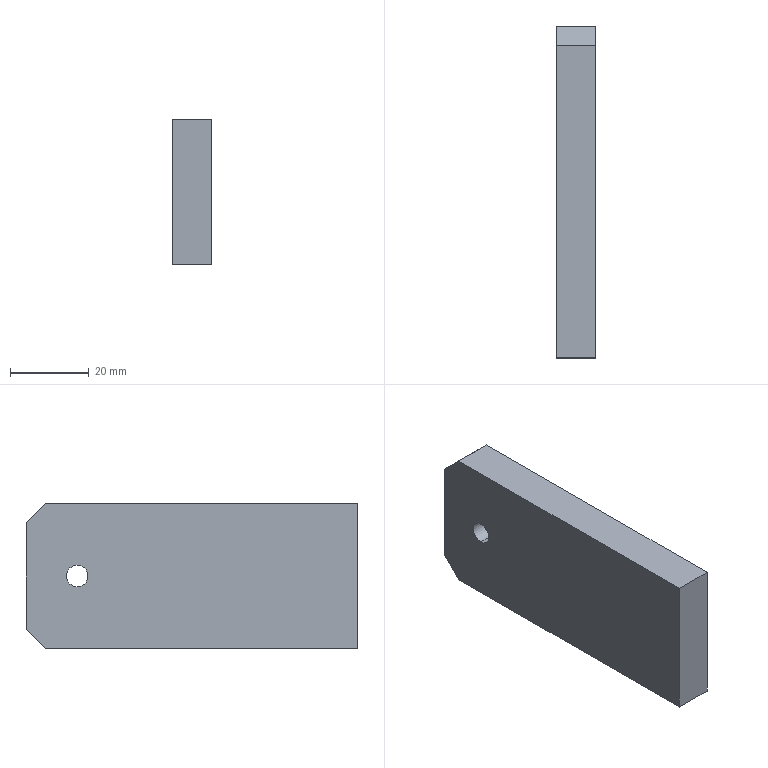Component | SolidWorks | AS-011-JG0134-1 | 1 solid | 10 faces | box 10 x 84.5 x 37 mm | volume 30777 mm3 | plane 8 | cylinder 2 | commonest cylinder face diameters 5.5 x2
build123d program:
from build123d import *

# Parameters (mm, degrees)
SKETCH1_R           = 2.75
BOSS_EXTRUDE1_DEPTH = 10


with BuildPart() as part:
    # Sketch1 → Boss-Extrude1 (new body)
    with BuildSketch(Plane.XY):
        Polygon((-18.5, -5), (-18.5, -84.5), (18.5, -84.5), (18.5, -5), (13.5, 0), (-13.5, 0), align=None)
        with Locations((0, -13)):
            Circle(SKETCH1_R, mode=Mode.SUBTRACT)
    extrude(amount=BOSS_EXTRUDE1_DEPTH)


solid = part.part

# Placed as in the assembly
solid = solid.moved(Location((-61.5, -15, -112), (0, 90, 0)))
STEP:
#1=COLOUR_RGB('',0.7922,0.8196,0.9333);
#2=FILL_AREA_STYLE_COLOUR('',#1);
#3=FILL_AREA_STYLE('',(#2));
#4=SURFACE_STYLE_FILL_AREA(#3);
#5=SURFACE_SIDE_STYLE('',(#4));
#6=SURFACE_STYLE_USAGE(.BOTH.,#5);
#7=PRESENTATION_STYLE_ASSIGNMENT((#6));
#8=CARTESIAN_POINT('',(-2.028,-1.102,-4.301));
#9=VERTEX_POINT('',#8);
#10=CARTESIAN_POINT('',(-2.028,-1.102,-4.518));
#11=VERTEX_POINT('',#10);
#12=CARTESIAN_POINT('',(-2.028,-1.102,-4.409));
#13=DIRECTION('',(1.,-0.,-0.));
#14=DIRECTION('',(-0.,0.,-1.));
#15=AXIS2_PLACEMENT_3D('',#12,#13,#14);
#16=CIRCLE('',#15,0.1083);
#17=EDGE_CURVE('',#9,#11,#16,.T.);
#18=ORIENTED_EDGE('',*,*,#17,.T.);
#19=CARTESIAN_POINT('',(-2.421,-1.102,-4.518));
#20=VERTEX_POINT('',#19);
#21=CARTESIAN_POINT('',(-2.028,-1.102,-4.518));
#22=DIRECTION('',(-1.,0.,0.));
#23=VECTOR('',#22,39.37);
#24=LINE('',#21,#23);
#25=EDGE_CURVE('',#11,#20,#24,.T.);
#26=ORIENTED_EDGE('',*,*,#25,.T.);
#27=CARTESIAN_POINT('',(-2.421,-1.102,-4.301));
#28=VERTEX_POINT('',#27);
#29=CARTESIAN_POINT('',(-2.421,-1.102,-4.409));
#30=DIRECTION('',(1.,-0.,-0.));
#31=DIRECTION('',(-0.,0.,-1.));
#32=AXIS2_PLACEMENT_3D('',#29,#30,#31);
#33=CIRCLE('',#32,0.1083);
#34=EDGE_CURVE('',#28,#20,#33,.T.);
#35=ORIENTED_EDGE('',*,*,#34,.F.);
#36=CARTESIAN_POINT('',(-2.028,-1.102,-4.301));
#37=DIRECTION('',(-1.,0.,0.));
#38=VECTOR('',#37,39.37);
#39=LINE('',#36,#38);
#40=EDGE_CURVE('',#9,#28,#39,.T.);
#41=ORIENTED_EDGE('',*,*,#40,.F.);
#42=EDGE_LOOP('',(#18,#26,#35,#41));
#43=FACE_OUTER_BOUND('',#42,.T.);
#44=CARTESIAN_POINT('',(-2.028,-1.102,-4.409));
#45=DIRECTION('',(-1.,0.,0.));
#46=DIRECTION('',(0.,0.,1.));
#47=AXIS2_PLACEMENT_3D('',#44,#45,#46);
#48=CYLINDRICAL_SURFACE('',#47,0.1083);
#49=ADVANCED_FACE('',(#43),#48,.F.);
#50=CARTESIAN_POINT('',(-2.028,-0.7874,-3.681));
#51=VERTEX_POINT('',#50);
#52=CARTESIAN_POINT('',(-2.028,-0.5906,-3.878));
#53=VERTEX_POINT('',#52);
#54=CARTESIAN_POINT('',(-2.028,-0.7874,-3.681));
#55=DIRECTION('',(-0.,0.7071,-0.7071));
#56=VECTOR('',#55,39.37);
#57=LINE('',#54,#56);
#58=EDGE_CURVE('',#51,#53,#57,.T.);
#59=ORIENTED_EDGE('',*,*,#58,.F.);
#60=CARTESIAN_POINT('',(-2.028,-3.917,-3.681));
#61=VERTEX_POINT('',#60);
#62=CARTESIAN_POINT('',(-2.028,-0.7874,-3.681));
#63=DIRECTION('',(-0.,-1.,0.));
#64=VECTOR('',#63,39.37);
#65=LINE('',#62,#64);
#66=EDGE_CURVE('',#51,#61,#65,.T.);
#67=ORIENTED_EDGE('',*,*,#66,.T.);
#68=CARTESIAN_POINT('',(-2.028,-3.917,-5.138));
#69=VERTEX_POINT('',#68);
#70=CARTESIAN_POINT('',(-2.028,-3.917,-3.681));
#71=DIRECTION('',(-0.,-0.,-1.));
#72=VECTOR('',#71,39.37);
#73=LINE('',#70,#72);
#74=EDGE_CURVE('',#61,#69,#73,.T.);
#75=ORIENTED_EDGE('',*,*,#74,.T.);
#76=CARTESIAN_POINT('',(-2.028,-0.7874,-5.138));
#77=VERTEX_POINT('',#76);
#78=CARTESIAN_POINT('',(-2.028,-0.7874,-5.138));
#79=DIRECTION('',(-0.,-1.,0.));
#80=VECTOR('',#79,39.37);
#81=LINE('',#78,#80);
#82=EDGE_CURVE('',#77,#69,#81,.T.);
#83=ORIENTED_EDGE('',*,*,#82,.F.);
#84=CARTESIAN_POINT('',(-2.028,-0.5906,-4.941));
#85=VERTEX_POINT('',#84);
#86=CARTESIAN_POINT('',(-2.028,-0.5906,-4.941));
#87=DIRECTION('',(-0.,-0.7071,-0.7071));
#88=VECTOR('',#87,39.37);
#89=LINE('',#86,#88);
#90=EDGE_CURVE('',#85,#77,#89,.T.);
#91=ORIENTED_EDGE('',*,*,#90,.F.);
#92=CARTESIAN_POINT('',(-2.028,-0.5906,-3.878));
#93=DIRECTION('',(-0.,-0.,-1.));
#94=VECTOR('',#93,39.37);
#95=LINE('',#92,#94);
#96=EDGE_CURVE('',#53,#85,#95,.T.);
#97=ORIENTED_EDGE('',*,*,#96,.F.);
#98=EDGE_LOOP('',(#59,#67,#75,#83,#91,#97));
#99=FACE_OUTER_BOUND('',#98,.T.);
#100=ORIENTED_EDGE('',*,*,#17,.F.);
#101=CARTESIAN_POINT('',(-2.028,-1.102,-4.409));
#102=DIRECTION('',(1.,-0.,-0.));
#103=DIRECTION('',(-0.,0.,-1.));
#104=AXIS2_PLACEMENT_3D('',#101,#102,#103);
#105=CIRCLE('',#104,0.1083);
#106=EDGE_CURVE('',#11,#9,#105,.T.);
#107=ORIENTED_EDGE('',*,*,#106,.F.);
#108=EDGE_LOOP('',(#100,#107));
#109=FACE_BOUND('',#108,.T.);
#110=CARTESIAN_POINT('',(-2.028,-0.5906,-4.409));
#111=DIRECTION('',(-1.,0.,0.));
#112=DIRECTION('',(0.,0.,1.));
#113=AXIS2_PLACEMENT_3D('',#110,#111,#112);
#114=PLANE('',#113);
#115=ADVANCED_FACE('',(#99,#109),#114,.F.);
#116=CARTESIAN_POINT('',(-2.421,-0.7874,-3.681));
#117=VERTEX_POINT('',#116);
#118=CARTESIAN_POINT('',(-2.421,-0.5906,-3.878));
#119=VERTEX_POINT('',#118);
#120=CARTESIAN_POINT('',(-2.421,-0.7874,-3.681));
#121=DIRECTION('',(-0.,0.7071,-0.7071));
#122=VECTOR('',#121,39.37);
#123=LINE('',#120,#122);
#124=EDGE_CURVE('',#117,#119,#123,.T.);
#125=ORIENTED_EDGE('',*,*,#124,.T.);
#126=CARTESIAN_POINT('',(-2.421,-0.5906,-4.941));
#127=VERTEX_POINT('',#126);
#128=CARTESIAN_POINT('',(-2.421,-0.5906,-3.878));
#129=DIRECTION('',(-0.,-0.,-1.));
#130=VECTOR('',#129,39.37);
#131=LINE('',#128,#130);
#132=EDGE_CURVE('',#119,#127,#131,.T.);
#133=ORIENTED_EDGE('',*,*,#132,.T.);
#134=CARTESIAN_POINT('',(-2.421,-0.7874,-5.138));
#135=VERTEX_POINT('',#134);
#136=CARTESIAN_POINT('',(-2.421,-0.5906,-4.941));
#137=DIRECTION('',(-0.,-0.7071,-0.7071));
#138=VECTOR('',#137,39.37);
#139=LINE('',#136,#138);
#140=EDGE_CURVE('',#127,#135,#139,.T.);
#141=ORIENTED_EDGE('',*,*,#140,.T.);
#142=CARTESIAN_POINT('',(-2.421,-3.917,-5.138));
#143=VERTEX_POINT('',#142);
#144=CARTESIAN_POINT('',(-2.421,-0.7874,-5.138));
#145=DIRECTION('',(-0.,-1.,0.));
#146=VECTOR('',#145,39.37);
#147=LINE('',#144,#146);
#148=EDGE_CURVE('',#135,#143,#147,.T.);
#149=ORIENTED_EDGE('',*,*,#148,.T.);
#150=CARTESIAN_POINT('',(-2.421,-3.917,-3.681));
#151=VERTEX_POINT('',#150);
#152=CARTESIAN_POINT('',(-2.421,-3.917,-3.681));
#153=DIRECTION('',(-0.,-0.,-1.));
#154=VECTOR('',#153,39.37);
#155=LINE('',#152,#154);
#156=EDGE_CURVE('',#151,#143,#155,.T.);
#157=ORIENTED_EDGE('',*,*,#156,.F.);
#158=CARTESIAN_POINT('',(-2.421,-0.7874,-3.681));
#159=DIRECTION('',(-0.,-1.,0.));
#160=VECTOR('',#159,39.37);
#161=LINE('',#158,#160);
#162=EDGE_CURVE('',#117,#151,#161,.T.);
#163=ORIENTED_EDGE('',*,*,#162,.F.);
#164=EDGE_LOOP('',(#125,#133,#141,#149,#157,#163));
#165=FACE_OUTER_BOUND('',#164,.T.);
#166=ORIENTED_EDGE('',*,*,#34,.T.);
#167=CARTESIAN_POINT('',(-2.421,-1.102,-4.409));
#168=DIRECTION('',(1.,-0.,-0.));
#169=DIRECTION('',(-0.,0.,-1.));
#170=AXIS2_PLACEMENT_3D('',#167,#168,#169);
#171=CIRCLE('',#170,0.1083);
#172=EDGE_CURVE('',#20,#28,#171,.T.);
#173=ORIENTED_EDGE('',*,*,#172,.T.);
#174=EDGE_LOOP('',(#166,#173));
#175=FACE_BOUND('',#174,.T.);
#176=CARTESIAN_POINT('',(-2.421,-0.5906,-4.409));
#177=DIRECTION('',(-1.,0.,0.));
#178=DIRECTION('',(0.,0.,1.));
#179=AXIS2_PLACEMENT_3D('',#176,#177,#178);
#180=PLANE('',#179);
#181=ADVANCED_FACE('',(#165,#175),#180,.T.);
#182=ORIENTED_EDGE('',*,*,#124,.F.);
#183=CARTESIAN_POINT('',(-2.028,-0.7874,-3.681));
#184=DIRECTION('',(-1.,0.,0.));
#185=VECTOR('',#184,39.37);
#186=LINE('',#183,#185);
#187=EDGE_CURVE('',#51,#117,#186,.T.);
#188=ORIENTED_EDGE('',*,*,#187,.F.);
#189=ORIENTED_EDGE('',*,*,#58,.T.);
#190=CARTESIAN_POINT('',(-2.028,-0.5906,-3.878));
#191=DIRECTION('',(-1.,0.,0.));
#192=VECTOR('',#191,39.37);
#193=LINE('',#190,#192);
#194=EDGE_CURVE('',#53,#119,#193,.T.);
#195=ORIENTED_EDGE('',*,*,#194,.T.);
#196=EDGE_LOOP('',(#182,#188,#189,#195));
#197=FACE_OUTER_BOUND('',#196,.T.);
#198=CARTESIAN_POINT('',(-2.028,-0.7874,-3.681));
#199=DIRECTION('',(0.,0.7071,0.7071));
#200=DIRECTION('',(0.,-0.7071,0.7071));
#201=AXIS2_PLACEMENT_3D('',#198,#199,#200);
#202=PLANE('',#201);
#203=ADVANCED_FACE('',(#197),#202,.T.);
#204=ORIENTED_EDGE('',*,*,#162,.T.);
#205=CARTESIAN_POINT('',(-2.028,-3.917,-3.681));
#206=DIRECTION('',(-1.,0.,0.));
#207=VECTOR('',#206,39.37);
#208=LINE('',#205,#207);
#209=EDGE_CURVE('',#61,#151,#208,.T.);
#210=ORIENTED_EDGE('',*,*,#209,.F.);
#211=ORIENTED_EDGE('',*,*,#66,.F.);
#212=ORIENTED_EDGE('',*,*,#187,.T.);
#213=EDGE_LOOP('',(#204,#210,#211,#212));
#214=FACE_OUTER_BOUND('',#213,.T.);
#215=CARTESIAN_POINT('',(-2.028,-0.7874,-3.681));
#216=DIRECTION('',(-0.,-0.,-1.));
#217=DIRECTION('',(-1.,0.,0.));
#218=AXIS2_PLACEMENT_3D('',#215,#216,#217);
#219=PLANE('',#218);
#220=ADVANCED_FACE('',(#214),#219,.F.);
#221=ORIENTED_EDGE('',*,*,#156,.T.);
#222=CARTESIAN_POINT('',(-2.028,-3.917,-5.138));
#223=DIRECTION('',(-1.,0.,0.));
#224=VECTOR('',#223,39.37);
#225=LINE('',#222,#224);
#226=EDGE_CURVE('',#69,#143,#225,.T.);
#227=ORIENTED_EDGE('',*,*,#226,.F.);
#228=ORIENTED_EDGE('',*,*,#74,.F.);
#229=ORIENTED_EDGE('',*,*,#209,.T.);
#230=EDGE_LOOP('',(#221,#227,#228,#229));
#231=FACE_OUTER_BOUND('',#230,.T.);
#232=CARTESIAN_POINT('',(-2.028,-3.917,-3.681));
#233=DIRECTION('',(0.,1.,-0.));
#234=DIRECTION('',(1.,-0.,-0.));
#235=AXIS2_PLACEMENT_3D('',#232,#233,#234);
#236=PLANE('',#235);
#237=ADVANCED_FACE('',(#231),#236,.F.);
#238=ORIENTED_EDGE('',*,*,#148,.F.);
#239=CARTESIAN_POINT('',(-2.028,-0.7874,-5.138));
#240=DIRECTION('',(-1.,0.,0.));
#241=VECTOR('',#240,39.37);
#242=LINE('',#239,#241);
#243=EDGE_CURVE('',#77,#135,#242,.T.);
#244=ORIENTED_EDGE('',*,*,#243,.F.);
#245=ORIENTED_EDGE('',*,*,#82,.T.);
#246=ORIENTED_EDGE('',*,*,#226,.T.);
#247=EDGE_LOOP('',(#238,#244,#245,#246));
#248=FACE_OUTER_BOUND('',#247,.T.);
#249=CARTESIAN_POINT('',(-2.028,-0.7874,-5.138));
#250=DIRECTION('',(-0.,-0.,-1.));
#251=DIRECTION('',(-1.,0.,0.));
#252=AXIS2_PLACEMENT_3D('',#249,#250,#251);
#253=PLANE('',#252);
#254=ADVANCED_FACE('',(#248),#253,.T.);
#255=ORIENTED_EDGE('',*,*,#140,.F.);
#256=CARTESIAN_POINT('',(-2.028,-0.5906,-4.941));
#257=DIRECTION('',(-1.,0.,0.));
#258=VECTOR('',#257,39.37);
#259=LINE('',#256,#258);
#260=EDGE_CURVE('',#85,#127,#259,.T.);
#261=ORIENTED_EDGE('',*,*,#260,.F.);
#262=ORIENTED_EDGE('',*,*,#90,.T.);
#263=ORIENTED_EDGE('',*,*,#243,.T.);
#264=EDGE_LOOP('',(#255,#261,#262,#263));
#265=FACE_OUTER_BOUND('',#264,.T.);
#266=CARTESIAN_POINT('',(-2.028,-0.5906,-4.941));
#267=DIRECTION('',(-0.,0.7071,-0.7071));
#268=DIRECTION('',(0.,0.7071,0.7071));
#269=AXIS2_PLACEMENT_3D('',#266,#267,#268);
#270=PLANE('',#269);
#271=ADVANCED_FACE('',(#265),#270,.T.);
#272=ORIENTED_EDGE('',*,*,#132,.F.);
#273=ORIENTED_EDGE('',*,*,#194,.F.);
#274=ORIENTED_EDGE('',*,*,#96,.T.);
#275=ORIENTED_EDGE('',*,*,#260,.T.);
#276=EDGE_LOOP('',(#272,#273,#274,#275));
#277=FACE_OUTER_BOUND('',#276,.T.);
#278=CARTESIAN_POINT('',(-2.028,-0.5906,-3.878));
#279=DIRECTION('',(0.,1.,-0.));
#280=DIRECTION('',(1.,-0.,-0.));
#281=AXIS2_PLACEMENT_3D('',#278,#279,#280);
#282=PLANE('',#281);
#283=ADVANCED_FACE('',(#277),#282,.T.);
#284=ORIENTED_EDGE('',*,*,#25,.F.);
#285=ORIENTED_EDGE('',*,*,#106,.T.);
#286=ORIENTED_EDGE('',*,*,#40,.T.);
#287=ORIENTED_EDGE('',*,*,#172,.F.);
#288=EDGE_LOOP('',(#284,#285,#286,#287));
#289=FACE_OUTER_BOUND('',#288,.T.);
#290=CARTESIAN_POINT('',(-2.028,-1.102,-4.409));
#291=DIRECTION('',(-1.,0.,0.));
#292=DIRECTION('',(0.,0.,1.));
#293=AXIS2_PLACEMENT_3D('',#290,#291,#292);
#294=CYLINDRICAL_SURFACE('',#293,0.1083);
#295=ADVANCED_FACE('',(#289),#294,.F.);
#296=CLOSED_SHELL('',(#49,#115,#181,#203,#220,#237,#254,#271,#283,#295));
#297=MANIFOLD_SOLID_BREP('',#296);
#298=STYLED_ITEM('',(#7),#297);
#299=PRESENTATION_LAYER_ASSIGNMENT('','',(#298));
#300=CARTESIAN_POINT('',(0.,0.,0.));
#301=DIRECTION('',(0.,0.,1.));
#302=DIRECTION('',(1.,0.,0.));
#303=AXIS2_PLACEMENT_3D('',#300,#301,#302);
#304=(LENGTH_UNIT()NAMED_UNIT(*)SI_UNIT($,.METRE.));
#305=LENGTH_MEASURE_WITH_UNIT(LENGTH_MEASURE(0.0254),#304);
#306=DIMENSIONAL_EXPONENTS(1.,0.,0.,0.,0.,0.,0.);
#307=(CONVERSION_BASED_UNIT('',#305)LENGTH_UNIT()NAMED_UNIT(#306));
#308=UNCERTAINTY_MEASURE_WITH_UNIT(LENGTH_MEASURE(0.00001),#307,'','');
#309=(NAMED_UNIT(*)PLANE_ANGLE_UNIT()SI_UNIT($,.RADIAN.));
#310=(NAMED_UNIT(*)SI_UNIT($,.STERADIAN.)SOLID_ANGLE_UNIT());
#311=(GEOMETRIC_REPRESENTATION_CONTEXT(3)GLOBAL_UNCERTAINTY_ASSIGNED_CONTEXT((#308))GLOBAL_UNIT_ASSIGNED_CONTEXT((#307,#309,#310))REPRESENTATION_CONTEXT('',''));
#312=ADVANCED_BREP_SHAPE_REPRESENTATION('',(#297,#303),#311);
#313=(LENGTH_UNIT()NAMED_UNIT(*)SI_UNIT($,.METRE.));
#314=LENGTH_MEASURE_WITH_UNIT(LENGTH_MEASURE(0.0254),#313);
#315=DIMENSIONAL_EXPONENTS(1.,0.,0.,0.,0.,0.,0.);
#316=(CONVERSION_BASED_UNIT('',#314)LENGTH_UNIT()NAMED_UNIT(#315));
#317=UNCERTAINTY_MEASURE_WITH_UNIT(LENGTH_MEASURE(0.00001),#316,'','');
#318=(NAMED_UNIT(*)PLANE_ANGLE_UNIT()SI_UNIT($,.RADIAN.));
#319=(NAMED_UNIT(*)SI_UNIT($,.STERADIAN.)SOLID_ANGLE_UNIT());
#320=(GEOMETRIC_REPRESENTATION_CONTEXT(3)GLOBAL_UNCERTAINTY_ASSIGNED_CONTEXT((#317))GLOBAL_UNIT_ASSIGNED_CONTEXT((#316,#318,#319))REPRESENTATION_CONTEXT('',''));
#321=MECHANICAL_DESIGN_GEOMETRIC_PRESENTATION_REPRESENTATION('',(#298),#320);